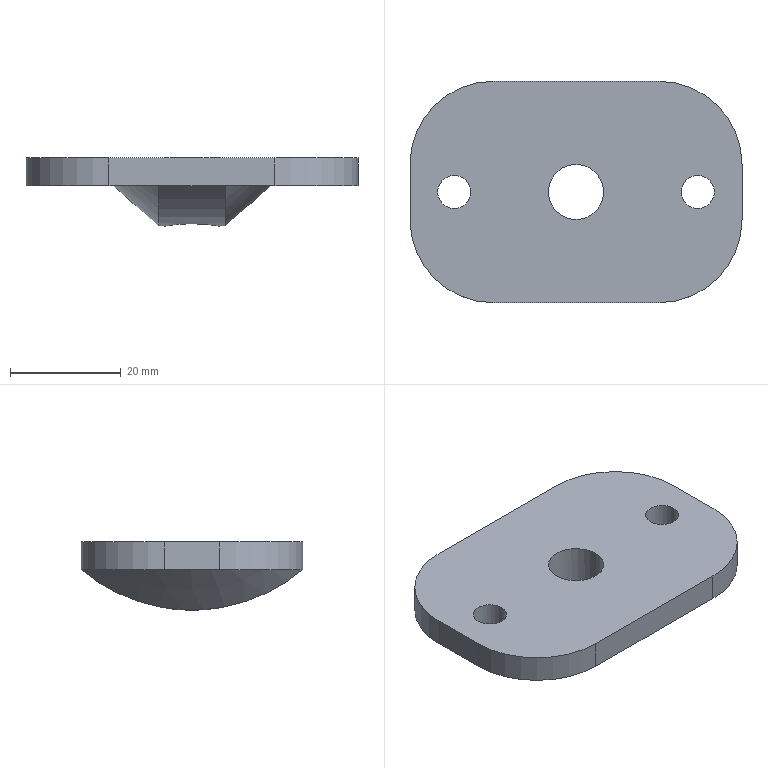Component | SolidWorks | AssemblyVibratoryFeederChassis-1_AssemblyWheel-1_WheelRetainingBlock-1 | 1 solid | 20 faces | box 60 x 40 x 12.34 mm | volume 13492 mm3 | cylinder 11 | plane 7 | cone 2 | commonest cylinder face diameters 6 x4 30 x4 10 x2 61.852 x1
STEP:
#1=COLOUR_RGB('',0.7922,0.8196,0.9333);
#2=FILL_AREA_STYLE_COLOUR('',#1);
#3=FILL_AREA_STYLE('',(#2));
#4=SURFACE_STYLE_FILL_AREA(#3);
#5=SURFACE_SIDE_STYLE('',(#4));
#6=SURFACE_STYLE_USAGE(.BOTH.,#5);
#7=PRESENTATION_STYLE_ASSIGNMENT((#6));
#8=CARTESIAN_POINT('',(-10.175,-11.07,-3.031));
#9=VERTEX_POINT('',#8);
#10=CARTESIAN_POINT('',(-9.939,-11.07,-3.031));
#11=VERTEX_POINT('',#10);
#12=CARTESIAN_POINT('',(-10.057,-11.07,-3.031));
#13=DIRECTION('',(0.,0.,1.));
#14=DIRECTION('',(1.,0.,0.));
#15=AXIS2_PLACEMENT_3D('',#12,#13,#14);
#16=CIRCLE('',#15,0.1181);
#17=EDGE_CURVE('',#9,#11,#16,.T.);
#18=ORIENTED_EDGE('',*,*,#17,.F.);
#19=CARTESIAN_POINT('',(-10.175,-11.07,-2.835));
#20=VERTEX_POINT('',#19);
#21=CARTESIAN_POINT('',(-10.175,-11.07,-5.984));
#22=DIRECTION('',(0.,0.,1.));
#23=VECTOR('',#22,39.37);
#24=LINE('',#21,#23);
#25=EDGE_CURVE('',#9,#20,#24,.T.);
#26=ORIENTED_EDGE('',*,*,#25,.T.);
#27=CARTESIAN_POINT('',(-9.939,-11.07,-2.835));
#28=VERTEX_POINT('',#27);
#29=CARTESIAN_POINT('',(-10.057,-11.07,-2.835));
#30=DIRECTION('',(0.,0.,1.));
#31=DIRECTION('',(1.,0.,0.));
#32=AXIS2_PLACEMENT_3D('',#29,#30,#31);
#33=CIRCLE('',#32,0.1181);
#34=EDGE_CURVE('',#20,#28,#33,.T.);
#35=ORIENTED_EDGE('',*,*,#34,.T.);
#36=CARTESIAN_POINT('',(-9.939,-11.07,-5.984));
#37=DIRECTION('',(0.,0.,1.));
#38=VECTOR('',#37,39.37);
#39=LINE('',#36,#38);
#40=EDGE_CURVE('',#11,#28,#39,.T.);
#41=ORIENTED_EDGE('',*,*,#40,.F.);
#42=EDGE_LOOP('',(#18,#26,#35,#41));
#43=FACE_OUTER_BOUND('',#42,.T.);
#44=CARTESIAN_POINT('',(-10.057,-11.07,-5.984));
#45=DIRECTION('',(0.,0.,1.));
#46=DIRECTION('',(1.,0.,0.));
#47=AXIS2_PLACEMENT_3D('',#44,#45,#46);
#48=CYLINDRICAL_SURFACE('',#47,0.1181);
#49=ADVANCED_FACE('',(#43),#48,.F.);
#50=CARTESIAN_POINT('',(-11.907,-11.07,-3.031));
#51=VERTEX_POINT('',#50);
#52=CARTESIAN_POINT('',(-11.671,-11.07,-3.031));
#53=VERTEX_POINT('',#52);
#54=CARTESIAN_POINT('',(-11.789,-11.07,-3.031));
#55=DIRECTION('',(0.,0.,1.));
#56=DIRECTION('',(1.,0.,0.));
#57=AXIS2_PLACEMENT_3D('',#54,#55,#56);
#58=CIRCLE('',#57,0.1181);
#59=EDGE_CURVE('',#51,#53,#58,.T.);
#60=ORIENTED_EDGE('',*,*,#59,.F.);
#61=CARTESIAN_POINT('',(-11.907,-11.07,-2.835));
#62=VERTEX_POINT('',#61);
#63=CARTESIAN_POINT('',(-11.907,-11.07,-5.984));
#64=DIRECTION('',(0.,0.,1.));
#65=VECTOR('',#64,39.37);
#66=LINE('',#63,#65);
#67=EDGE_CURVE('',#51,#62,#66,.T.);
#68=ORIENTED_EDGE('',*,*,#67,.T.);
#69=CARTESIAN_POINT('',(-11.671,-11.07,-2.835));
#70=VERTEX_POINT('',#69);
#71=CARTESIAN_POINT('',(-11.789,-11.07,-2.835));
#72=DIRECTION('',(0.,0.,1.));
#73=DIRECTION('',(1.,0.,0.));
#74=AXIS2_PLACEMENT_3D('',#71,#72,#73);
#75=CIRCLE('',#74,0.1181);
#76=EDGE_CURVE('',#62,#70,#75,.T.);
#77=ORIENTED_EDGE('',*,*,#76,.T.);
#78=CARTESIAN_POINT('',(-11.671,-11.07,-5.984));
#79=DIRECTION('',(0.,0.,1.));
#80=VECTOR('',#79,39.37);
#81=LINE('',#78,#80);
#82=EDGE_CURVE('',#53,#70,#81,.T.);
#83=ORIENTED_EDGE('',*,*,#82,.F.);
#84=EDGE_LOOP('',(#60,#68,#77,#83));
#85=FACE_OUTER_BOUND('',#84,.T.);
#86=CARTESIAN_POINT('',(-11.789,-11.07,-5.984));
#87=DIRECTION('',(0.,0.,1.));
#88=DIRECTION('',(1.,0.,0.));
#89=AXIS2_PLACEMENT_3D('',#86,#87,#88);
#90=CYLINDRICAL_SURFACE('',#89,0.1181);
#91=ADVANCED_FACE('',(#85),#90,.F.);
#92=CARTESIAN_POINT('',(-10.726,-11.07,-3.32));
#93=VERTEX_POINT('',#92);
#94=CARTESIAN_POINT('',(-11.12,-11.07,-3.32));
#95=VERTEX_POINT('',#94);
#96=CARTESIAN_POINT('',(-10.726,-11.07,-3.32));
#97=CARTESIAN_POINT('',(-10.726,-11.083,-3.32));
#98=CARTESIAN_POINT('',(-10.728,-11.096,-3.32));
#99=CARTESIAN_POINT('',(-10.731,-11.115,-3.32));
#100=CARTESIAN_POINT('',(-10.733,-11.121,-3.319));
#101=CARTESIAN_POINT('',(-10.737,-11.133,-3.319));
#102=CARTESIAN_POINT('',(-10.739,-11.139,-3.318));
#103=CARTESIAN_POINT('',(-10.746,-11.157,-3.317));
#104=CARTESIAN_POINT('',(-10.752,-11.169,-3.316));
#105=CARTESIAN_POINT('',(-10.767,-11.19,-3.314));
#106=CARTESIAN_POINT('',(-10.775,-11.2,-3.313));
#107=CARTESIAN_POINT('',(-10.793,-11.218,-3.311));
#108=CARTESIAN_POINT('',(-10.803,-11.226,-3.31));
#109=CARTESIAN_POINT('',(-10.824,-11.241,-3.308));
#110=CARTESIAN_POINT('',(-10.836,-11.247,-3.307));
#111=CARTESIAN_POINT('',(-10.86,-11.257,-3.306));
#112=CARTESIAN_POINT('',(-10.872,-11.26,-3.305));
#113=CARTESIAN_POINT('',(-10.897,-11.266,-3.305));
#114=CARTESIAN_POINT('',(-10.91,-11.267,-3.304));
#115=CARTESIAN_POINT('',(-10.936,-11.267,-3.304));
#116=CARTESIAN_POINT('',(-10.949,-11.265,-3.305));
#117=CARTESIAN_POINT('',(-10.974,-11.26,-3.305));
#118=CARTESIAN_POINT('',(-10.987,-11.257,-3.306));
#119=CARTESIAN_POINT('',(-11.004,-11.249,-3.307));
#120=CARTESIAN_POINT('',(-11.01,-11.247,-3.308));
#121=CARTESIAN_POINT('',(-11.022,-11.24,-3.308));
#122=CARTESIAN_POINT('',(-11.027,-11.237,-3.309));
#123=CARTESIAN_POINT('',(-11.043,-11.226,-3.31));
#124=CARTESIAN_POINT('',(-11.053,-11.218,-3.311));
#125=CARTESIAN_POINT('',(-11.072,-11.2,-3.313));
#126=CARTESIAN_POINT('',(-11.08,-11.19,-3.314));
#127=CARTESIAN_POINT('',(-11.094,-11.169,-3.316));
#128=CARTESIAN_POINT('',(-11.1,-11.157,-3.317));
#129=CARTESIAN_POINT('',(-11.11,-11.133,-3.319));
#130=CARTESIAN_POINT('',(-11.114,-11.121,-3.319));
#131=CARTESIAN_POINT('',(-11.119,-11.096,-3.32));
#132=CARTESIAN_POINT('',(-11.12,-11.083,-3.32));
#133=CARTESIAN_POINT('',(-11.12,-11.07,-3.32));
#134=B_SPLINE_CURVE_WITH_KNOTS('',3,(#96,#97,#98,#99,#100,#101,#102,#103,#104,#105,#106,#107,#108,#109,#110,#111,#112,#113,#114,#115,#116,#117,#118,#119,#120,#121,#122,#123,#124,#125,#126,#127,#128,#129,#130,#131,#132,#133),.UNSPECIFIED.,.F.,.F.,(4,2,2,2,2,2,2,2,2,2,2,2,2,2,2,2,2,2,4),(0.,0.0009786,0.001468,0.001957,0.002936,0.003914,0.004893,0.005872,0.00685,0.007829,0.008808,0.009786,0.01028,0.01076,0.01174,0.01272,0.0137,0.01468,0.01566),.UNSPECIFIED.);
#135=EDGE_CURVE('',#93,#95,#134,.T.);
#136=ORIENTED_EDGE('',*,*,#135,.T.);
#137=CARTESIAN_POINT('',(-11.12,-11.07,-2.835));
#138=VERTEX_POINT('',#137);
#139=CARTESIAN_POINT('',(-11.12,-11.07,-3.32));
#140=DIRECTION('',(0.,0.,1.));
#141=VECTOR('',#140,39.37);
#142=LINE('',#139,#141);
#143=EDGE_CURVE('',#95,#138,#142,.T.);
#144=ORIENTED_EDGE('',*,*,#143,.T.);
#145=CARTESIAN_POINT('',(-10.726,-11.07,-2.835));
#146=VERTEX_POINT('',#145);
#147=CARTESIAN_POINT('',(-10.923,-11.07,-2.835));
#148=DIRECTION('',(0.,0.,1.));
#149=DIRECTION('',(1.,0.,0.));
#150=AXIS2_PLACEMENT_3D('',#147,#148,#149);
#151=CIRCLE('',#150,0.1969);
#152=EDGE_CURVE('',#138,#146,#151,.T.);
#153=ORIENTED_EDGE('',*,*,#152,.T.);
#154=CARTESIAN_POINT('',(-10.726,-11.07,-3.32));
#155=DIRECTION('',(0.,0.,1.));
#156=VECTOR('',#155,39.37);
#157=LINE('',#154,#156);
#158=EDGE_CURVE('',#93,#146,#157,.T.);
#159=ORIENTED_EDGE('',*,*,#158,.F.);
#160=EDGE_LOOP('',(#136,#144,#153,#159));
#161=FACE_OUTER_BOUND('',#160,.T.);
#162=CARTESIAN_POINT('',(-10.923,-11.07,-3.32));
#163=DIRECTION('',(0.,0.,1.));
#164=DIRECTION('',(1.,0.,0.));
#165=AXIS2_PLACEMENT_3D('',#162,#163,#164);
#166=CYLINDRICAL_SURFACE('',#165,0.1969);
#167=ADVANCED_FACE('',(#161),#166,.F.);
#168=ORIENTED_EDGE('',*,*,#135,.F.);
#169=CARTESIAN_POINT('',(-11.12,-11.07,-3.32));
#170=CARTESIAN_POINT('',(-11.12,-11.057,-3.32));
#171=CARTESIAN_POINT('',(-11.119,-11.044,-3.32));
#172=CARTESIAN_POINT('',(-11.114,-11.019,-3.319));
#173=CARTESIAN_POINT('',(-11.11,-11.006,-3.319));
#174=CARTESIAN_POINT('',(-11.1,-10.983,-3.317));
#175=CARTESIAN_POINT('',(-11.094,-10.971,-3.316));
#176=CARTESIAN_POINT('',(-11.08,-10.95,-3.314));
#177=CARTESIAN_POINT('',(-11.072,-10.94,-3.313));
#178=CARTESIAN_POINT('',(-11.053,-10.922,-3.311));
#179=CARTESIAN_POINT('',(-11.043,-10.913,-3.31));
#180=CARTESIAN_POINT('',(-11.022,-10.899,-3.308));
#181=CARTESIAN_POINT('',(-11.011,-10.893,-3.307));
#182=CARTESIAN_POINT('',(-10.993,-10.886,-3.306));
#183=CARTESIAN_POINT('',(-10.987,-10.883,-3.306));
#184=CARTESIAN_POINT('',(-10.974,-10.88,-3.305));
#185=CARTESIAN_POINT('',(-10.968,-10.878,-3.305));
#186=CARTESIAN_POINT('',(-10.949,-10.874,-3.305));
#187=CARTESIAN_POINT('',(-10.936,-10.873,-3.304));
#188=CARTESIAN_POINT('',(-10.91,-10.873,-3.304));
#189=CARTESIAN_POINT('',(-10.897,-10.874,-3.305));
#190=CARTESIAN_POINT('',(-10.872,-10.879,-3.305));
#191=CARTESIAN_POINT('',(-10.86,-10.883,-3.306));
#192=CARTESIAN_POINT('',(-10.836,-10.893,-3.307));
#193=CARTESIAN_POINT('',(-10.825,-10.899,-3.308));
#194=CARTESIAN_POINT('',(-10.803,-10.913,-3.31));
#195=CARTESIAN_POINT('',(-10.793,-10.922,-3.311));
#196=CARTESIAN_POINT('',(-10.775,-10.94,-3.313));
#197=CARTESIAN_POINT('',(-10.767,-10.95,-3.314));
#198=CARTESIAN_POINT('',(-10.752,-10.971,-3.316));
#199=CARTESIAN_POINT('',(-10.746,-10.982,-3.317));
#200=CARTESIAN_POINT('',(-10.736,-11.006,-3.319));
#201=CARTESIAN_POINT('',(-10.733,-11.019,-3.319));
#202=CARTESIAN_POINT('',(-10.728,-11.044,-3.32));
#203=CARTESIAN_POINT('',(-10.726,-11.057,-3.32));
#204=CARTESIAN_POINT('',(-10.726,-11.07,-3.32));
#205=B_SPLINE_CURVE_WITH_KNOTS('',3,(#169,#170,#171,#172,#173,#174,#175,#176,#177,#178,#179,#180,#181,#182,#183,#184,#185,#186,#187,#188,#189,#190,#191,#192,#193,#194,#195,#196,#197,#198,#199,#200,#201,#202,#203,#204),.UNSPECIFIED.,.F.,.F.,(4,2,2,2,2,2,2,2,2,2,2,2,2,2,2,2,2,4),(0.01566,0.01664,0.01761,0.01859,0.01957,0.02055,0.02153,0.02202,0.02251,0.02349,0.02446,0.02544,0.02642,0.0274,0.02838,0.02936,0.03033,0.03131),.UNSPECIFIED.);
#206=EDGE_CURVE('',#95,#93,#205,.T.);
#207=ORIENTED_EDGE('',*,*,#206,.F.);
#208=EDGE_LOOP('',(#168,#207));
#209=FACE_BOUND('',#208,.T.);
#210=CARTESIAN_POINT('',(-11.159,-11.857,-3.031));
#211=VERTEX_POINT('',#210);
#212=CARTESIAN_POINT('',(-10.687,-11.857,-3.031));
#213=VERTEX_POINT('',#212);
#214=CARTESIAN_POINT('',(-12.104,-11.857,-3.031));
#215=DIRECTION('',(1.,-0.,-0.));
#216=VECTOR('',#215,39.37);
#217=LINE('',#214,#216);
#218=EDGE_CURVE('',#211,#213,#217,.T.);
#219=ORIENTED_EDGE('',*,*,#218,.F.);
#220=CARTESIAN_POINT('',(-11.159,-10.283,-3.031));
#221=VERTEX_POINT('',#220);
#222=CARTESIAN_POINT('',(-11.159,-11.07,-2.103));
#223=DIRECTION('',(1.,-0.,-0.));
#224=DIRECTION('',(0.,1.,0.));
#225=AXIS2_PLACEMENT_3D('',#222,#223,#224);
#226=CIRCLE('',#225,1.218);
#227=EDGE_CURVE('',#211,#221,#226,.T.);
#228=ORIENTED_EDGE('',*,*,#227,.T.);
#229=CARTESIAN_POINT('',(-10.687,-10.283,-3.031));
#230=VERTEX_POINT('',#229);
#231=CARTESIAN_POINT('',(-12.104,-10.283,-3.031));
#232=DIRECTION('',(1.,-0.,-0.));
#233=VECTOR('',#232,39.37);
#234=LINE('',#231,#233);
#235=EDGE_CURVE('',#221,#230,#234,.T.);
#236=ORIENTED_EDGE('',*,*,#235,.T.);
#237=CARTESIAN_POINT('',(-10.687,-11.07,-2.103));
#238=DIRECTION('',(-1.,0.,0.));
#239=DIRECTION('',(0.,-1.,0.));
#240=AXIS2_PLACEMENT_3D('',#237,#238,#239);
#241=CIRCLE('',#240,1.218);
#242=EDGE_CURVE('',#230,#213,#241,.T.);
#243=ORIENTED_EDGE('',*,*,#242,.T.);
#244=EDGE_LOOP('',(#219,#228,#236,#243));
#245=FACE_OUTER_BOUND('',#244,.T.);
#246=CARTESIAN_POINT('',(-12.104,-11.07,-2.103));
#247=DIRECTION('',(1.,-0.,-0.));
#248=DIRECTION('',(0.,1.,0.));
#249=AXIS2_PLACEMENT_3D('',#246,#247,#248);
#250=CYLINDRICAL_SURFACE('',#249,1.218);
#251=ADVANCED_FACE('',(#209,#245),#250,.T.);
#252=CARTESIAN_POINT('',(-10.333,-11.857,-3.031));
#253=VERTEX_POINT('',#252);
#254=CARTESIAN_POINT('',(-9.742,-11.857,-3.031));
#255=DIRECTION('',(-1.,0.,0.));
#256=VECTOR('',#255,39.37);
#257=LINE('',#254,#256);
#258=EDGE_CURVE('',#253,#213,#257,.T.);
#259=ORIENTED_EDGE('',*,*,#258,.F.);
#260=CARTESIAN_POINT('',(-10.333,-11.857,-2.835));
#261=VERTEX_POINT('',#260);
#262=CARTESIAN_POINT('',(-10.333,-11.857,-2.835));
#263=DIRECTION('',(0.,0.,1.));
#264=VECTOR('',#263,39.37);
#265=LINE('',#262,#264);
#266=EDGE_CURVE('',#253,#261,#265,.T.);
#267=ORIENTED_EDGE('',*,*,#266,.T.);
#268=CARTESIAN_POINT('',(-11.514,-11.857,-2.835));
#269=VERTEX_POINT('',#268);
#270=CARTESIAN_POINT('',(-12.104,-11.857,-2.835));
#271=DIRECTION('',(1.,-0.,-0.));
#272=VECTOR('',#271,39.37);
#273=LINE('',#270,#272);
#274=EDGE_CURVE('',#269,#261,#273,.T.);
#275=ORIENTED_EDGE('',*,*,#274,.F.);
#276=CARTESIAN_POINT('',(-11.514,-11.857,-3.031));
#277=VERTEX_POINT('',#276);
#278=CARTESIAN_POINT('',(-11.514,-11.857,-3.031));
#279=DIRECTION('',(-0.,-0.,-1.));
#280=VECTOR('',#279,39.37);
#281=LINE('',#278,#280);
#282=EDGE_CURVE('',#269,#277,#281,.T.);
#283=ORIENTED_EDGE('',*,*,#282,.T.);
#284=CARTESIAN_POINT('',(-12.104,-11.857,-3.031));
#285=DIRECTION('',(1.,-0.,-0.));
#286=VECTOR('',#285,39.37);
#287=LINE('',#284,#286);
#288=EDGE_CURVE('',#277,#211,#287,.T.);
#289=ORIENTED_EDGE('',*,*,#288,.T.);
#290=ORIENTED_EDGE('',*,*,#218,.T.);
#291=EDGE_LOOP('',(#259,#267,#275,#283,#289,#290));
#292=FACE_OUTER_BOUND('',#291,.T.);
#293=CARTESIAN_POINT('',(-12.104,-11.857,-2.835));
#294=DIRECTION('',(-0.,-1.,0.));
#295=DIRECTION('',(1.,-0.,-0.));
#296=AXIS2_PLACEMENT_3D('',#293,#294,#295);
#297=PLANE('',#296);
#298=ADVANCED_FACE('',(#292),#297,.T.);
#299=CARTESIAN_POINT('',(-10.057,-11.07,-2.835));
#300=DIRECTION('',(0.,0.,1.));
#301=DIRECTION('',(1.,0.,0.));
#302=AXIS2_PLACEMENT_3D('',#299,#300,#301);
#303=CIRCLE('',#302,0.1181);
#304=EDGE_CURVE('',#28,#20,#303,.T.);
#305=ORIENTED_EDGE('',*,*,#304,.F.);
#306=ORIENTED_EDGE('',*,*,#34,.F.);
#307=EDGE_LOOP('',(#305,#306));
#308=FACE_BOUND('',#307,.T.);
#309=CARTESIAN_POINT('',(-11.789,-11.07,-2.835));
#310=DIRECTION('',(0.,0.,1.));
#311=DIRECTION('',(1.,0.,0.));
#312=AXIS2_PLACEMENT_3D('',#309,#310,#311);
#313=CIRCLE('',#312,0.1181);
#314=EDGE_CURVE('',#70,#62,#313,.T.);
#315=ORIENTED_EDGE('',*,*,#314,.F.);
#316=ORIENTED_EDGE('',*,*,#76,.F.);
#317=EDGE_LOOP('',(#315,#316));
#318=FACE_BOUND('',#317,.T.);
#319=CARTESIAN_POINT('',(-10.923,-11.07,-2.835));
#320=DIRECTION('',(0.,0.,1.));
#321=DIRECTION('',(1.,0.,0.));
#322=AXIS2_PLACEMENT_3D('',#319,#320,#321);
#323=CIRCLE('',#322,0.1969);
#324=EDGE_CURVE('',#146,#138,#323,.T.);
#325=ORIENTED_EDGE('',*,*,#324,.F.);
#326=ORIENTED_EDGE('',*,*,#152,.F.);
#327=EDGE_LOOP('',(#325,#326));
#328=FACE_BOUND('',#327,.T.);
#329=ORIENTED_EDGE('',*,*,#274,.T.);
#330=CARTESIAN_POINT('',(-9.742,-11.267,-2.835));
#331=VERTEX_POINT('',#330);
#332=CARTESIAN_POINT('',(-10.333,-11.267,-2.835));
#333=DIRECTION('',(0.,0.,1.));
#334=DIRECTION('',(1.,0.,0.));
#335=AXIS2_PLACEMENT_3D('',#332,#333,#334);
#336=CIRCLE('',#335,0.5906);
#337=EDGE_CURVE('',#261,#331,#336,.T.);
#338=ORIENTED_EDGE('',*,*,#337,.T.);
#339=CARTESIAN_POINT('',(-9.742,-10.873,-2.835));
#340=VERTEX_POINT('',#339);
#341=CARTESIAN_POINT('',(-9.742,-11.857,-2.835));
#342=DIRECTION('',(-0.,-1.,0.));
#343=VECTOR('',#342,39.37);
#344=LINE('',#341,#343);
#345=EDGE_CURVE('',#340,#331,#344,.T.);
#346=ORIENTED_EDGE('',*,*,#345,.F.);
#347=CARTESIAN_POINT('',(-10.333,-10.283,-2.835));
#348=VERTEX_POINT('',#347);
#349=CARTESIAN_POINT('',(-10.333,-10.873,-2.835));
#350=DIRECTION('',(0.,0.,1.));
#351=DIRECTION('',(1.,0.,0.));
#352=AXIS2_PLACEMENT_3D('',#349,#350,#351);
#353=CIRCLE('',#352,0.5906);
#354=EDGE_CURVE('',#340,#348,#353,.T.);
#355=ORIENTED_EDGE('',*,*,#354,.T.);
#356=CARTESIAN_POINT('',(-11.514,-10.283,-2.835));
#357=VERTEX_POINT('',#356);
#358=CARTESIAN_POINT('',(-12.104,-10.283,-2.835));
#359=DIRECTION('',(1.,-0.,-0.));
#360=VECTOR('',#359,39.37);
#361=LINE('',#358,#360);
#362=EDGE_CURVE('',#357,#348,#361,.T.);
#363=ORIENTED_EDGE('',*,*,#362,.F.);
#364=CARTESIAN_POINT('',(-12.104,-10.873,-2.835));
#365=VERTEX_POINT('',#364);
#366=CARTESIAN_POINT('',(-11.514,-10.873,-2.835));
#367=DIRECTION('',(0.,0.,1.));
#368=DIRECTION('',(1.,0.,0.));
#369=AXIS2_PLACEMENT_3D('',#366,#367,#368);
#370=CIRCLE('',#369,0.5906);
#371=EDGE_CURVE('',#357,#365,#370,.T.);
#372=ORIENTED_EDGE('',*,*,#371,.T.);
#373=CARTESIAN_POINT('',(-12.104,-11.267,-2.835));
#374=VERTEX_POINT('',#373);
#375=CARTESIAN_POINT('',(-12.104,-11.857,-2.835));
#376=DIRECTION('',(-0.,-1.,0.));
#377=VECTOR('',#376,39.37);
#378=LINE('',#375,#377);
#379=EDGE_CURVE('',#365,#374,#378,.T.);
#380=ORIENTED_EDGE('',*,*,#379,.T.);
#381=CARTESIAN_POINT('',(-11.514,-11.267,-2.835));
#382=DIRECTION('',(0.,0.,1.));
#383=DIRECTION('',(1.,0.,0.));
#384=AXIS2_PLACEMENT_3D('',#381,#382,#383);
#385=CIRCLE('',#384,0.5906);
#386=EDGE_CURVE('',#374,#269,#385,.T.);
#387=ORIENTED_EDGE('',*,*,#386,.T.);
#388=EDGE_LOOP('',(#329,#338,#346,#355,#363,#372,#380,#387));
#389=FACE_OUTER_BOUND('',#388,.T.);
#390=CARTESIAN_POINT('',(-12.104,-11.857,-2.835));
#391=DIRECTION('',(0.,0.,1.));
#392=DIRECTION('',(1.,-0.,-0.));
#393=AXIS2_PLACEMENT_3D('',#390,#391,#392);
#394=PLANE('',#393);
#395=ADVANCED_FACE('',(#308,#318,#328,#389),#394,.T.);
#396=ORIENTED_EDGE('',*,*,#362,.T.);
#397=CARTESIAN_POINT('',(-10.333,-10.283,-3.031));
#398=VERTEX_POINT('',#397);
#399=CARTESIAN_POINT('',(-10.333,-10.283,-2.835));
#400=DIRECTION('',(-0.,-0.,-1.));
#401=VECTOR('',#400,39.37);
#402=LINE('',#399,#401);
#403=EDGE_CURVE('',#348,#398,#402,.T.);
#404=ORIENTED_EDGE('',*,*,#403,.T.);
#405=CARTESIAN_POINT('',(-9.742,-10.283,-3.031));
#406=DIRECTION('',(-1.,0.,0.));
#407=VECTOR('',#406,39.37);
#408=LINE('',#405,#407);
#409=EDGE_CURVE('',#398,#230,#408,.T.);
#410=ORIENTED_EDGE('',*,*,#409,.T.);
#411=ORIENTED_EDGE('',*,*,#235,.F.);
#412=CARTESIAN_POINT('',(-11.514,-10.283,-3.031));
#413=VERTEX_POINT('',#412);
#414=CARTESIAN_POINT('',(-12.104,-10.283,-3.031));
#415=DIRECTION('',(1.,-0.,-0.));
#416=VECTOR('',#415,39.37);
#417=LINE('',#414,#416);
#418=EDGE_CURVE('',#413,#221,#417,.T.);
#419=ORIENTED_EDGE('',*,*,#418,.F.);
#420=CARTESIAN_POINT('',(-11.514,-10.283,-2.835));
#421=DIRECTION('',(0.,0.,1.));
#422=VECTOR('',#421,39.37);
#423=LINE('',#420,#422);
#424=EDGE_CURVE('',#413,#357,#423,.T.);
#425=ORIENTED_EDGE('',*,*,#424,.T.);
#426=EDGE_LOOP('',(#396,#404,#410,#411,#419,#425));
#427=FACE_OUTER_BOUND('',#426,.T.);
#428=CARTESIAN_POINT('',(-12.104,-10.283,-2.835));
#429=DIRECTION('',(0.,1.,-0.));
#430=DIRECTION('',(-1.,0.,0.));
#431=AXIS2_PLACEMENT_3D('',#428,#429,#430);
#432=PLANE('',#431);
#433=ADVANCED_FACE('',(#427),#432,.T.);
#434=ORIENTED_EDGE('',*,*,#379,.F.);
#435=CARTESIAN_POINT('',(-12.104,-10.873,-3.031));
#436=VERTEX_POINT('',#435);
#437=CARTESIAN_POINT('',(-12.104,-10.873,-3.031));
#438=DIRECTION('',(-0.,-0.,-1.));
#439=VECTOR('',#438,39.37);
#440=LINE('',#437,#439);
#441=EDGE_CURVE('',#365,#436,#440,.T.);
#442=ORIENTED_EDGE('',*,*,#441,.T.);
#443=CARTESIAN_POINT('',(-12.104,-11.267,-3.031));
#444=VERTEX_POINT('',#443);
#445=CARTESIAN_POINT('',(-12.104,-10.283,-3.031));
#446=DIRECTION('',(-0.,-1.,0.));
#447=VECTOR('',#446,39.37);
#448=LINE('',#445,#447);
#449=EDGE_CURVE('',#436,#444,#448,.T.);
#450=ORIENTED_EDGE('',*,*,#449,.T.);
#451=CARTESIAN_POINT('',(-12.104,-11.267,-2.835));
#452=DIRECTION('',(0.,0.,1.));
#453=VECTOR('',#452,39.37);
#454=LINE('',#451,#453);
#455=EDGE_CURVE('',#444,#374,#454,.T.);
#456=ORIENTED_EDGE('',*,*,#455,.T.);
#457=EDGE_LOOP('',(#434,#442,#450,#456));
#458=FACE_OUTER_BOUND('',#457,.T.);
#459=CARTESIAN_POINT('',(-12.104,-11.07,-2.103));
#460=DIRECTION('',(1.,-0.,-0.));
#461=DIRECTION('',(0.,1.,-0.));
#462=AXIS2_PLACEMENT_3D('',#459,#460,#461);
#463=PLANE('',#462);
#464=ADVANCED_FACE('',(#458),#463,.F.);
#465=ORIENTED_EDGE('',*,*,#345,.T.);
#466=CARTESIAN_POINT('',(-9.742,-11.267,-3.031));
#467=VERTEX_POINT('',#466);
#468=CARTESIAN_POINT('',(-9.742,-11.267,-2.103));
#469=DIRECTION('',(-0.,-0.,-1.));
#470=VECTOR('',#469,39.37);
#471=LINE('',#468,#470);
#472=EDGE_CURVE('',#331,#467,#471,.T.);
#473=ORIENTED_EDGE('',*,*,#472,.T.);
#474=CARTESIAN_POINT('',(-9.742,-10.873,-3.031));
#475=VERTEX_POINT('',#474);
#476=CARTESIAN_POINT('',(-9.742,-10.283,-3.031));
#477=DIRECTION('',(-0.,-1.,0.));
#478=VECTOR('',#477,39.37);
#479=LINE('',#476,#478);
#480=EDGE_CURVE('',#475,#467,#479,.T.);
#481=ORIENTED_EDGE('',*,*,#480,.F.);
#482=CARTESIAN_POINT('',(-9.742,-10.873,-2.103));
#483=DIRECTION('',(0.,0.,1.));
#484=VECTOR('',#483,39.37);
#485=LINE('',#482,#484);
#486=EDGE_CURVE('',#475,#340,#485,.T.);
#487=ORIENTED_EDGE('',*,*,#486,.T.);
#488=EDGE_LOOP('',(#465,#473,#481,#487));
#489=FACE_OUTER_BOUND('',#488,.T.);
#490=CARTESIAN_POINT('',(-9.742,-11.07,-2.103));
#491=DIRECTION('',(1.,-0.,-0.));
#492=DIRECTION('',(0.,1.,-0.));
#493=AXIS2_PLACEMENT_3D('',#490,#491,#492);
#494=PLANE('',#493);
#495=ADVANCED_FACE('',(#489),#494,.T.);
#496=CARTESIAN_POINT('',(-11.789,-11.07,-3.031));
#497=DIRECTION('',(0.,0.,1.));
#498=DIRECTION('',(1.,0.,0.));
#499=AXIS2_PLACEMENT_3D('',#496,#497,#498);
#500=CIRCLE('',#499,0.1181);
#501=EDGE_CURVE('',#53,#51,#500,.T.);
#502=ORIENTED_EDGE('',*,*,#501,.T.);
#503=ORIENTED_EDGE('',*,*,#59,.T.);
#504=EDGE_LOOP('',(#502,#503));
#505=FACE_BOUND('',#504,.T.);
#506=ORIENTED_EDGE('',*,*,#449,.F.);
#507=CARTESIAN_POINT('',(-11.514,-10.873,-3.031));
#508=DIRECTION('',(-0.,-0.,-1.));
#509=DIRECTION('',(1.,0.,0.));
#510=AXIS2_PLACEMENT_3D('',#507,#508,#509);
#511=CIRCLE('',#510,0.5906);
#512=EDGE_CURVE('',#436,#413,#511,.T.);
#513=ORIENTED_EDGE('',*,*,#512,.T.);
#514=ORIENTED_EDGE('',*,*,#418,.T.);
#515=CARTESIAN_POINT('',(-11.159,-10.283,-3.031));
#516=CARTESIAN_POINT('',(-11.202,-10.341,-3.031));
#517=CARTESIAN_POINT('',(-11.243,-10.4,-3.031));
#518=CARTESIAN_POINT('',(-11.318,-10.523,-3.031));
#519=CARTESIAN_POINT('',(-11.353,-10.586,-3.031));
#520=CARTESIAN_POINT('',(-11.391,-10.668,-3.031));
#521=CARTESIAN_POINT('',(-11.398,-10.684,-3.031));
#522=CARTESIAN_POINT('',(-11.412,-10.718,-3.031));
#523=CARTESIAN_POINT('',(-11.418,-10.734,-3.031));
#524=CARTESIAN_POINT('',(-11.437,-10.786,-3.031));
#525=CARTESIAN_POINT('',(-11.448,-10.82,-3.031));
#526=CARTESIAN_POINT('',(-11.466,-10.89,-3.031));
#527=CARTESIAN_POINT('',(-11.472,-10.925,-3.031));
#528=CARTESIAN_POINT('',(-11.48,-10.979,-3.031));
#529=CARTESIAN_POINT('',(-11.481,-10.997,-3.031));
#530=CARTESIAN_POINT('',(-11.484,-11.033,-3.031));
#531=CARTESIAN_POINT('',(-11.484,-11.051,-3.031));
#532=CARTESIAN_POINT('',(-11.484,-11.105,-3.031));
#533=CARTESIAN_POINT('',(-11.482,-11.142,-3.031));
#534=CARTESIAN_POINT('',(-11.475,-11.195,-3.031));
#535=CARTESIAN_POINT('',(-11.472,-11.213,-3.031));
#536=CARTESIAN_POINT('',(-11.465,-11.249,-3.031));
#537=CARTESIAN_POINT('',(-11.461,-11.267,-3.031));
#538=CARTESIAN_POINT('',(-11.439,-11.355,-3.031));
#539=CARTESIAN_POINT('',(-11.414,-11.422,-3.031));
#540=CARTESIAN_POINT('',(-11.369,-11.52,-3.031));
#541=CARTESIAN_POINT('',(-11.353,-11.552,-3.031));
#542=CARTESIAN_POINT('',(-11.318,-11.615,-3.031));
#543=CARTESIAN_POINT('',(-11.3,-11.647,-3.031));
#544=CARTESIAN_POINT('',(-11.243,-11.739,-3.031));
#545=CARTESIAN_POINT('',(-11.202,-11.799,-3.031));
#546=CARTESIAN_POINT('',(-11.159,-11.857,-3.031));
#547=B_SPLINE_CURVE_WITH_KNOTS('',3,(#515,#516,#517,#518,#519,#520,#521,#522,#523,#524,#525,#526,#527,#528,#529,#530,#531,#532,#533,#534,#535,#536,#537,#538,#539,#540,#541,#542,#543,#544,#545,#546),.UNSPECIFIED.,.F.,.F.,(4,2,2,2,2,2,2,2,2,2,2,2,2,2,2,4),(-0.02659,-0.02112,-0.01565,-0.01428,-0.01291,-0.01018,-0.00744,-0.006072,-0.004704,-0.001969,-0.0006008,0.0007669,0.006238,0.008974,0.01171,0.01718),.UNSPECIFIED.);
#548=EDGE_CURVE('',#221,#211,#547,.T.);
#549=ORIENTED_EDGE('',*,*,#548,.T.);
#550=ORIENTED_EDGE('',*,*,#288,.F.);
#551=CARTESIAN_POINT('',(-11.514,-11.267,-3.031));
#552=DIRECTION('',(-0.,-0.,-1.));
#553=DIRECTION('',(1.,0.,0.));
#554=AXIS2_PLACEMENT_3D('',#551,#552,#553);
#555=CIRCLE('',#554,0.5906);
#556=EDGE_CURVE('',#277,#444,#555,.T.);
#557=ORIENTED_EDGE('',*,*,#556,.T.);
#558=EDGE_LOOP('',(#506,#513,#514,#549,#550,#557));
#559=FACE_OUTER_BOUND('',#558,.T.);
#560=CARTESIAN_POINT('',(-12.104,-10.283,-3.031));
#561=DIRECTION('',(0.,0.,1.));
#562=DIRECTION('',(1.,-0.,-0.));
#563=AXIS2_PLACEMENT_3D('',#560,#561,#562);
#564=PLANE('',#563);
#565=ADVANCED_FACE('',(#505,#559),#564,.F.);
#566=CARTESIAN_POINT('',(-10.057,-11.07,-3.031));
#567=DIRECTION('',(0.,0.,1.));
#568=DIRECTION('',(1.,0.,0.));
#569=AXIS2_PLACEMENT_3D('',#566,#567,#568);
#570=CIRCLE('',#569,0.1181);
#571=EDGE_CURVE('',#11,#9,#570,.T.);
#572=ORIENTED_EDGE('',*,*,#571,.T.);
#573=ORIENTED_EDGE('',*,*,#17,.T.);
#574=EDGE_LOOP('',(#572,#573));
#575=FACE_BOUND('',#574,.T.);
#576=ORIENTED_EDGE('',*,*,#480,.T.);
#577=CARTESIAN_POINT('',(-10.333,-11.267,-3.031));
#578=DIRECTION('',(-0.,-0.,-1.));
#579=DIRECTION('',(1.,0.,0.));
#580=AXIS2_PLACEMENT_3D('',#577,#578,#579);
#581=CIRCLE('',#580,0.5906);
#582=EDGE_CURVE('',#467,#253,#581,.T.);
#583=ORIENTED_EDGE('',*,*,#582,.T.);
#584=ORIENTED_EDGE('',*,*,#258,.T.);
#585=CARTESIAN_POINT('',(-10.687,-11.857,-3.031));
#586=CARTESIAN_POINT('',(-10.644,-11.799,-3.031));
#587=CARTESIAN_POINT('',(-10.604,-11.739,-3.031));
#588=CARTESIAN_POINT('',(-10.528,-11.617,-3.031));
#589=CARTESIAN_POINT('',(-10.494,-11.554,-3.031));
#590=CARTESIAN_POINT('',(-10.456,-11.472,-3.031));
#591=CARTESIAN_POINT('',(-10.448,-11.456,-3.031));
#592=CARTESIAN_POINT('',(-10.435,-11.422,-3.031));
#593=CARTESIAN_POINT('',(-10.428,-11.405,-3.031));
#594=CARTESIAN_POINT('',(-10.409,-11.354,-3.031));
#595=CARTESIAN_POINT('',(-10.398,-11.32,-3.031));
#596=CARTESIAN_POINT('',(-10.381,-11.25,-3.031));
#597=CARTESIAN_POINT('',(-10.374,-11.215,-3.031));
#598=CARTESIAN_POINT('',(-10.367,-11.161,-3.031));
#599=CARTESIAN_POINT('',(-10.365,-11.143,-3.031));
#600=CARTESIAN_POINT('',(-10.363,-11.107,-3.031));
#601=CARTESIAN_POINT('',(-10.362,-11.089,-3.031));
#602=CARTESIAN_POINT('',(-10.362,-11.034,-3.031));
#603=CARTESIAN_POINT('',(-10.364,-10.998,-3.031));
#604=CARTESIAN_POINT('',(-10.371,-10.945,-3.031));
#605=CARTESIAN_POINT('',(-10.374,-10.927,-3.031));
#606=CARTESIAN_POINT('',(-10.381,-10.891,-3.031));
#607=CARTESIAN_POINT('',(-10.385,-10.873,-3.031));
#608=CARTESIAN_POINT('',(-10.407,-10.785,-3.031));
#609=CARTESIAN_POINT('',(-10.432,-10.718,-3.031));
#610=CARTESIAN_POINT('',(-10.478,-10.62,-3.031));
#611=CARTESIAN_POINT('',(-10.494,-10.588,-3.031));
#612=CARTESIAN_POINT('',(-10.528,-10.525,-3.031));
#613=CARTESIAN_POINT('',(-10.547,-10.493,-3.031));
#614=CARTESIAN_POINT('',(-10.604,-10.401,-3.031));
#615=CARTESIAN_POINT('',(-10.644,-10.341,-3.031));
#616=CARTESIAN_POINT('',(-10.687,-10.283,-3.031));
#617=B_SPLINE_CURVE_WITH_KNOTS('',3,(#585,#586,#587,#588,#589,#590,#591,#592,#593,#594,#595,#596,#597,#598,#599,#600,#601,#602,#603,#604,#605,#606,#607,#608,#609,#610,#611,#612,#613,#614,#615,#616),.UNSPECIFIED.,.F.,.F.,(4,2,2,2,2,2,2,2,2,2,2,2,2,2,2,4),(-0.02659,-0.02112,-0.01565,-0.01428,-0.01291,-0.01018,-0.00744,-0.006072,-0.004704,-0.001969,-0.0006008,0.0007669,0.006238,0.008974,0.01171,0.01718),.UNSPECIFIED.);
#618=EDGE_CURVE('',#213,#230,#617,.T.);
#619=ORIENTED_EDGE('',*,*,#618,.T.);
#620=ORIENTED_EDGE('',*,*,#409,.F.);
#621=CARTESIAN_POINT('',(-10.333,-10.873,-3.031));
#622=DIRECTION('',(-0.,-0.,-1.));
#623=DIRECTION('',(1.,0.,0.));
#624=AXIS2_PLACEMENT_3D('',#621,#622,#623);
#625=CIRCLE('',#624,0.5906);
#626=EDGE_CURVE('',#398,#475,#625,.T.);
#627=ORIENTED_EDGE('',*,*,#626,.T.);
#628=EDGE_LOOP('',(#576,#583,#584,#619,#620,#627));
#629=FACE_OUTER_BOUND('',#628,.T.);
#630=CARTESIAN_POINT('',(-9.742,-10.283,-3.031));
#631=DIRECTION('',(0.,0.,1.));
#632=DIRECTION('',(1.,-0.,-0.));
#633=AXIS2_PLACEMENT_3D('',#630,#631,#632);
#634=PLANE('',#633);
#635=ADVANCED_FACE('',(#575,#629),#634,.F.);
#636=ORIENTED_EDGE('',*,*,#143,.F.);
#637=ORIENTED_EDGE('',*,*,#206,.T.);
#638=ORIENTED_EDGE('',*,*,#158,.T.);
#639=ORIENTED_EDGE('',*,*,#324,.T.);
#640=EDGE_LOOP('',(#636,#637,#638,#639));
#641=FACE_OUTER_BOUND('',#640,.T.);
#642=CARTESIAN_POINT('',(-10.923,-11.07,-3.32));
#643=DIRECTION('',(0.,0.,1.));
#644=DIRECTION('',(1.,0.,0.));
#645=AXIS2_PLACEMENT_3D('',#642,#643,#644);
#646=CYLINDRICAL_SURFACE('',#645,0.1969);
#647=ADVANCED_FACE('',(#641),#646,.F.);
#648=ORIENTED_EDGE('',*,*,#548,.F.);
#649=ORIENTED_EDGE('',*,*,#227,.F.);
#650=EDGE_LOOP('',(#648,#649));
#651=FACE_OUTER_BOUND('',#650,.T.);
#652=CARTESIAN_POINT('',(-11.514,-11.07,-2.103));
#653=DIRECTION('',(1.,-0.,-0.));
#654=DIRECTION('',(0.,1.,0.));
#655=AXIS2_PLACEMENT_3D('',#652,#653,#654);
#656=CONICAL_SURFACE('',#655,0.9026,0.7266);
#657=ADVANCED_FACE('',(#651),#656,.T.);
#658=ORIENTED_EDGE('',*,*,#618,.F.);
#659=ORIENTED_EDGE('',*,*,#242,.F.);
#660=EDGE_LOOP('',(#658,#659));
#661=FACE_OUTER_BOUND('',#660,.T.);
#662=CARTESIAN_POINT('',(-10.333,-11.07,-2.103));
#663=DIRECTION('',(-1.,0.,0.));
#664=DIRECTION('',(0.,-1.,0.));
#665=AXIS2_PLACEMENT_3D('',#662,#663,#664);
#666=CONICAL_SURFACE('',#665,0.9026,0.7266);
#667=ADVANCED_FACE('',(#661),#666,.T.);
#668=ORIENTED_EDGE('',*,*,#337,.F.);
#669=ORIENTED_EDGE('',*,*,#266,.F.);
#670=ORIENTED_EDGE('',*,*,#582,.F.);
#671=ORIENTED_EDGE('',*,*,#472,.F.);
#672=EDGE_LOOP('',(#668,#669,#670,#671));
#673=FACE_OUTER_BOUND('',#672,.T.);
#674=CARTESIAN_POINT('',(-10.333,-11.267,-2.103));
#675=DIRECTION('',(-0.,-0.,-1.));
#676=DIRECTION('',(-1.,0.,0.));
#677=AXIS2_PLACEMENT_3D('',#674,#675,#676);
#678=CYLINDRICAL_SURFACE('',#677,0.5906);
#679=ADVANCED_FACE('',(#673),#678,.T.);
#680=ORIENTED_EDGE('',*,*,#626,.F.);
#681=ORIENTED_EDGE('',*,*,#403,.F.);
#682=ORIENTED_EDGE('',*,*,#354,.F.);
#683=ORIENTED_EDGE('',*,*,#486,.F.);
#684=EDGE_LOOP('',(#680,#681,#682,#683));
#685=FACE_OUTER_BOUND('',#684,.T.);
#686=CARTESIAN_POINT('',(-10.333,-10.873,-2.103));
#687=DIRECTION('',(0.,0.,1.));
#688=DIRECTION('',(1.,0.,0.));
#689=AXIS2_PLACEMENT_3D('',#686,#687,#688);
#690=CYLINDRICAL_SURFACE('',#689,0.5906);
#691=ADVANCED_FACE('',(#685),#690,.T.);
#692=ORIENTED_EDGE('',*,*,#512,.F.);
#693=ORIENTED_EDGE('',*,*,#441,.F.);
#694=ORIENTED_EDGE('',*,*,#371,.F.);
#695=ORIENTED_EDGE('',*,*,#424,.F.);
#696=EDGE_LOOP('',(#692,#693,#694,#695));
#697=FACE_OUTER_BOUND('',#696,.T.);
#698=CARTESIAN_POINT('',(-11.514,-10.873,-2.835));
#699=DIRECTION('',(-0.,-0.,-1.));
#700=DIRECTION('',(-1.,0.,0.));
#701=AXIS2_PLACEMENT_3D('',#698,#699,#700);
#702=CYLINDRICAL_SURFACE('',#701,0.5906);
#703=ADVANCED_FACE('',(#697),#702,.T.);
#704=ORIENTED_EDGE('',*,*,#386,.F.);
#705=ORIENTED_EDGE('',*,*,#455,.F.);
#706=ORIENTED_EDGE('',*,*,#556,.F.);
#707=ORIENTED_EDGE('',*,*,#282,.F.);
#708=EDGE_LOOP('',(#704,#705,#706,#707));
#709=FACE_OUTER_BOUND('',#708,.T.);
#710=CARTESIAN_POINT('',(-11.514,-11.267,-2.835));
#711=DIRECTION('',(0.,0.,1.));
#712=DIRECTION('',(1.,0.,0.));
#713=AXIS2_PLACEMENT_3D('',#710,#711,#712);
#714=CYLINDRICAL_SURFACE('',#713,0.5906);
#715=ADVANCED_FACE('',(#709),#714,.T.);
#716=ORIENTED_EDGE('',*,*,#67,.F.);
#717=ORIENTED_EDGE('',*,*,#501,.F.);
#718=ORIENTED_EDGE('',*,*,#82,.T.);
#719=ORIENTED_EDGE('',*,*,#314,.T.);
#720=EDGE_LOOP('',(#716,#717,#718,#719));
#721=FACE_OUTER_BOUND('',#720,.T.);
#722=CARTESIAN_POINT('',(-11.789,-11.07,-5.984));
#723=DIRECTION('',(0.,0.,1.));
#724=DIRECTION('',(1.,0.,0.));
#725=AXIS2_PLACEMENT_3D('',#722,#723,#724);
#726=CYLINDRICAL_SURFACE('',#725,0.1181);
#727=ADVANCED_FACE('',(#721),#726,.F.);
#728=ORIENTED_EDGE('',*,*,#25,.F.);
#729=ORIENTED_EDGE('',*,*,#571,.F.);
#730=ORIENTED_EDGE('',*,*,#40,.T.);
#731=ORIENTED_EDGE('',*,*,#304,.T.);
#732=EDGE_LOOP('',(#728,#729,#730,#731));
#733=FACE_OUTER_BOUND('',#732,.T.);
#734=CARTESIAN_POINT('',(-10.057,-11.07,-5.984));
#735=DIRECTION('',(0.,0.,1.));
#736=DIRECTION('',(1.,0.,0.));
#737=AXIS2_PLACEMENT_3D('',#734,#735,#736);
#738=CYLINDRICAL_SURFACE('',#737,0.1181);
#739=ADVANCED_FACE('',(#733),#738,.F.);
#740=CLOSED_SHELL('',(#49,#91,#167,#251,#298,#395,#433,#464,#495,#565,#635,#647,#657,#667,#679,#691,#703,#715,#727,#739));
#741=MANIFOLD_SOLID_BREP('',#740);
#742=STYLED_ITEM('',(#7),#741);
#743=PRESENTATION_LAYER_ASSIGNMENT('','',(#742));
#744=CARTESIAN_POINT('',(0.,0.,0.));
#745=DIRECTION('',(0.,0.,1.));
#746=DIRECTION('',(1.,0.,0.));
#747=AXIS2_PLACEMENT_3D('',#744,#745,#746);
#748=(LENGTH_UNIT()NAMED_UNIT(*)SI_UNIT($,.METRE.));
#749=LENGTH_MEASURE_WITH_UNIT(LENGTH_MEASURE(0.0254),#748);
#750=DIMENSIONAL_EXPONENTS(1.,0.,0.,0.,0.,0.,0.);
#751=(CONVERSION_BASED_UNIT('',#749)LENGTH_UNIT()NAMED_UNIT(#750));
#752=UNCERTAINTY_MEASURE_WITH_UNIT(LENGTH_MEASURE(0.00001),#751,'','');
#753=(NAMED_UNIT(*)PLANE_ANGLE_UNIT()SI_UNIT($,.RADIAN.));
#754=(NAMED_UNIT(*)SI_UNIT($,.STERADIAN.)SOLID_ANGLE_UNIT());
#755=(GEOMETRIC_REPRESENTATION_CONTEXT(3)GLOBAL_UNCERTAINTY_ASSIGNED_CONTEXT((#752))GLOBAL_UNIT_ASSIGNED_CONTEXT((#751,#753,#754))REPRESENTATION_CONTEXT('',''));
#756=ADVANCED_BREP_SHAPE_REPRESENTATION('',(#741,#747),#755);
#757=(LENGTH_UNIT()NAMED_UNIT(*)SI_UNIT($,.METRE.));
#758=LENGTH_MEASURE_WITH_UNIT(LENGTH_MEASURE(0.0254),#757);
#759=DIMENSIONAL_EXPONENTS(1.,0.,0.,0.,0.,0.,0.);
#760=(CONVERSION_BASED_UNIT('',#758)LENGTH_UNIT()NAMED_UNIT(#759));
#761=UNCERTAINTY_MEASURE_WITH_UNIT(LENGTH_MEASURE(0.00001),#760,'','');
#762=(NAMED_UNIT(*)PLANE_ANGLE_UNIT()SI_UNIT($,.RADIAN.));
#763=(NAMED_UNIT(*)SI_UNIT($,.STERADIAN.)SOLID_ANGLE_UNIT());
#764=(GEOMETRIC_REPRESENTATION_CONTEXT(3)GLOBAL_UNCERTAINTY_ASSIGNED_CONTEXT((#761))GLOBAL_UNIT_ASSIGNED_CONTEXT((#760,#762,#763))REPRESENTATION_CONTEXT('',''));
#765=MECHANICAL_DESIGN_GEOMETRIC_PRESENTATION_REPRESENTATION('',(#742),#764);